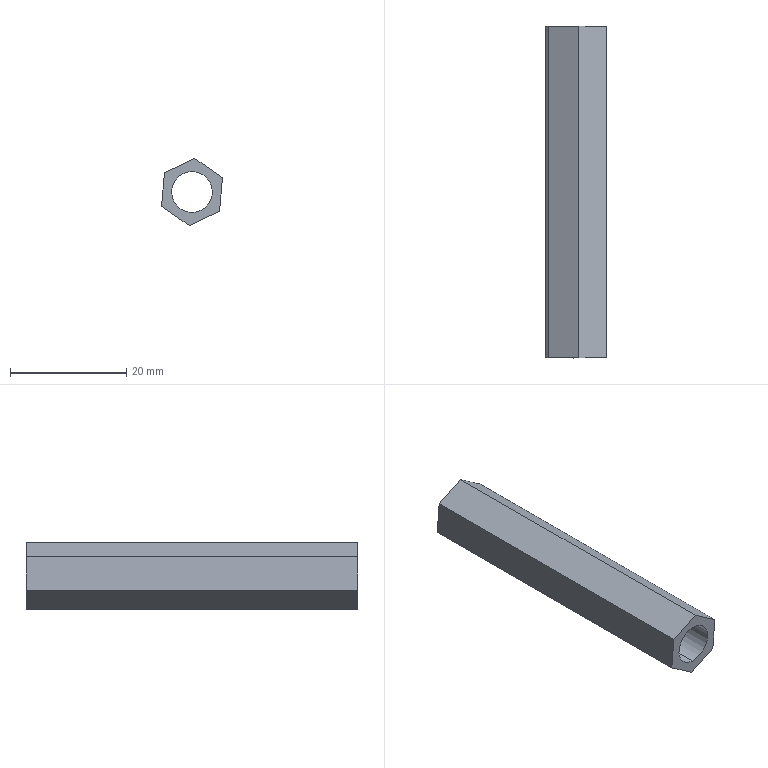Component | SolidWorks | HexagonalPost-1 | 1 solid | 10 faces | box 10.46 x 57 x 11.5 mm | volume 2743 mm3 | plane 8 | cylinder 2 | commonest cylinder face diameters 7 x2 | material Plain Carbon Steel
STEP:
#1=COLOUR_RGB('',0.7922,0.8196,0.9333);
#2=FILL_AREA_STYLE_COLOUR('',#1);
#3=FILL_AREA_STYLE('',(#2));
#4=SURFACE_STYLE_FILL_AREA(#3);
#5=SURFACE_SIDE_STYLE('',(#4));
#6=SURFACE_STYLE_USAGE(.BOTH.,#5);
#7=PRESENTATION_STYLE_ASSIGNMENT((#6));
#8=CARTESIAN_POINT('',(-177.617,347.975,291.332));
#9=VERTEX_POINT('',#8);
#10=CARTESIAN_POINT('',(-177.64,347.975,291.057));
#11=VERTEX_POINT('',#10);
#12=CARTESIAN_POINT('',(-177.628,347.975,291.195));
#13=DIRECTION('',(0.,1.,0.));
#14=DIRECTION('',(-0.08306,0.,-0.9965));
#15=AXIS2_PLACEMENT_3D('',#12,#13,#14);
#16=CIRCLE('',#15,0.1378);
#17=EDGE_CURVE('',#9,#11,#16,.T.);
#18=ORIENTED_EDGE('',*,*,#17,.T.);
#19=CARTESIAN_POINT('',(-177.64,345.731,291.057));
#20=VERTEX_POINT('',#19);
#21=CARTESIAN_POINT('',(-177.64,347.975,291.057));
#22=DIRECTION('',(-0.,-1.,-0.));
#23=VECTOR('',#22,39.37);
#24=LINE('',#21,#23);
#25=EDGE_CURVE('',#11,#20,#24,.T.);
#26=ORIENTED_EDGE('',*,*,#25,.T.);
#27=CARTESIAN_POINT('',(-177.617,345.731,291.332));
#28=VERTEX_POINT('',#27);
#29=CARTESIAN_POINT('',(-177.628,345.731,291.195));
#30=DIRECTION('',(0.,1.,0.));
#31=DIRECTION('',(-0.08306,0.,-0.9965));
#32=AXIS2_PLACEMENT_3D('',#29,#30,#31);
#33=CIRCLE('',#32,0.1378);
#34=EDGE_CURVE('',#28,#20,#33,.T.);
#35=ORIENTED_EDGE('',*,*,#34,.F.);
#36=CARTESIAN_POINT('',(-177.617,347.975,291.332));
#37=DIRECTION('',(-0.,-1.,-0.));
#38=VECTOR('',#37,39.37);
#39=LINE('',#36,#38);
#40=EDGE_CURVE('',#9,#28,#39,.T.);
#41=ORIENTED_EDGE('',*,*,#40,.F.);
#42=EDGE_LOOP('',(#18,#26,#35,#41));
#43=FACE_OUTER_BOUND('',#42,.T.);
#44=CARTESIAN_POINT('',(-177.628,347.975,291.195));
#45=DIRECTION('',(-0.,-1.,-0.));
#46=DIRECTION('',(0.08306,0.,0.9965));
#47=AXIS2_PLACEMENT_3D('',#44,#45,#46);
#48=CYLINDRICAL_SURFACE('',#47,0.1378);
#49=ADVANCED_FACE('',(#43),#48,.F.);
#50=CARTESIAN_POINT('',(-177.648,347.975,290.968));
#51=VERTEX_POINT('',#50);
#52=CARTESIAN_POINT('',(-177.834,347.975,291.098));
#53=VERTEX_POINT('',#52);
#54=CARTESIAN_POINT('',(-177.648,347.975,290.968));
#55=DIRECTION('',(-0.8199,0.,0.5726));
#56=VECTOR('',#55,39.37);
#57=LINE('',#54,#56);
#58=EDGE_CURVE('',#51,#53,#57,.T.);
#59=ORIENTED_EDGE('',*,*,#58,.T.);
#60=CARTESIAN_POINT('',(-177.815,347.975,291.325));
#61=VERTEX_POINT('',#60);
#62=CARTESIAN_POINT('',(-177.834,347.975,291.098));
#63=DIRECTION('',(0.08592,-0.,0.9963));
#64=VECTOR('',#63,39.37);
#65=LINE('',#62,#64);
#66=EDGE_CURVE('',#53,#61,#65,.T.);
#67=ORIENTED_EDGE('',*,*,#66,.T.);
#68=CARTESIAN_POINT('',(-177.609,347.975,291.421));
#69=VERTEX_POINT('',#68);
#70=CARTESIAN_POINT('',(-177.815,347.975,291.325));
#71=DIRECTION('',(0.9058,-0.,0.4237));
#72=VECTOR('',#71,39.37);
#73=LINE('',#70,#72);
#74=EDGE_CURVE('',#61,#69,#73,.T.);
#75=ORIENTED_EDGE('',*,*,#74,.T.);
#76=CARTESIAN_POINT('',(-177.422,347.975,291.291));
#77=VERTEX_POINT('',#76);
#78=CARTESIAN_POINT('',(-177.609,347.975,291.421));
#79=DIRECTION('',(0.8199,-0.,-0.5726));
#80=VECTOR('',#79,39.37);
#81=LINE('',#78,#80);
#82=EDGE_CURVE('',#69,#77,#81,.T.);
#83=ORIENTED_EDGE('',*,*,#82,.T.);
#84=CARTESIAN_POINT('',(-177.442,347.975,291.064));
#85=VERTEX_POINT('',#84);
#86=CARTESIAN_POINT('',(-177.422,347.975,291.291));
#87=DIRECTION('',(-0.08592,0.,-0.9963));
#88=VECTOR('',#87,39.37);
#89=LINE('',#86,#88);
#90=EDGE_CURVE('',#77,#85,#89,.T.);
#91=ORIENTED_EDGE('',*,*,#90,.T.);
#92=CARTESIAN_POINT('',(-177.442,347.975,291.064));
#93=DIRECTION('',(-0.9058,0.,-0.4237));
#94=VECTOR('',#93,39.37);
#95=LINE('',#92,#94);
#96=EDGE_CURVE('',#85,#51,#95,.T.);
#97=ORIENTED_EDGE('',*,*,#96,.T.);
#98=EDGE_LOOP('',(#59,#67,#75,#83,#91,#97));
#99=FACE_OUTER_BOUND('',#98,.T.);
#100=ORIENTED_EDGE('',*,*,#17,.F.);
#101=CARTESIAN_POINT('',(-177.628,347.975,291.195));
#102=DIRECTION('',(0.,1.,0.));
#103=DIRECTION('',(-0.08306,0.,-0.9965));
#104=AXIS2_PLACEMENT_3D('',#101,#102,#103);
#105=CIRCLE('',#104,0.1378);
#106=EDGE_CURVE('',#11,#9,#105,.T.);
#107=ORIENTED_EDGE('',*,*,#106,.F.);
#108=EDGE_LOOP('',(#100,#107));
#109=FACE_BOUND('',#108,.T.);
#110=CARTESIAN_POINT('',(-177.834,347.975,291.098));
#111=DIRECTION('',(0.,1.,0.));
#112=DIRECTION('',(-0.08306,0.,-0.9965));
#113=AXIS2_PLACEMENT_3D('',#110,#111,#112);
#114=PLANE('',#113);
#115=ADVANCED_FACE('',(#99,#109),#114,.T.);
#116=CARTESIAN_POINT('',(-177.648,345.731,290.968));
#117=VERTEX_POINT('',#116);
#118=CARTESIAN_POINT('',(-177.834,345.731,291.098));
#119=VERTEX_POINT('',#118);
#120=CARTESIAN_POINT('',(-177.648,345.731,290.968));
#121=DIRECTION('',(-0.8199,0.,0.5726));
#122=VECTOR('',#121,39.37);
#123=LINE('',#120,#122);
#124=EDGE_CURVE('',#117,#119,#123,.T.);
#125=ORIENTED_EDGE('',*,*,#124,.F.);
#126=CARTESIAN_POINT('',(-177.442,345.731,291.064));
#127=VERTEX_POINT('',#126);
#128=CARTESIAN_POINT('',(-177.442,345.731,291.064));
#129=DIRECTION('',(-0.9058,0.,-0.4237));
#130=VECTOR('',#129,39.37);
#131=LINE('',#128,#130);
#132=EDGE_CURVE('',#127,#117,#131,.T.);
#133=ORIENTED_EDGE('',*,*,#132,.F.);
#134=CARTESIAN_POINT('',(-177.422,345.731,291.291));
#135=VERTEX_POINT('',#134);
#136=CARTESIAN_POINT('',(-177.422,345.731,291.291));
#137=DIRECTION('',(-0.08592,0.,-0.9963));
#138=VECTOR('',#137,39.37);
#139=LINE('',#136,#138);
#140=EDGE_CURVE('',#135,#127,#139,.T.);
#141=ORIENTED_EDGE('',*,*,#140,.F.);
#142=CARTESIAN_POINT('',(-177.609,345.731,291.421));
#143=VERTEX_POINT('',#142);
#144=CARTESIAN_POINT('',(-177.609,345.731,291.421));
#145=DIRECTION('',(0.8199,-0.,-0.5726));
#146=VECTOR('',#145,39.37);
#147=LINE('',#144,#146);
#148=EDGE_CURVE('',#143,#135,#147,.T.);
#149=ORIENTED_EDGE('',*,*,#148,.F.);
#150=CARTESIAN_POINT('',(-177.815,345.731,291.325));
#151=VERTEX_POINT('',#150);
#152=CARTESIAN_POINT('',(-177.815,345.731,291.325));
#153=DIRECTION('',(0.9058,-0.,0.4237));
#154=VECTOR('',#153,39.37);
#155=LINE('',#152,#154);
#156=EDGE_CURVE('',#151,#143,#155,.T.);
#157=ORIENTED_EDGE('',*,*,#156,.F.);
#158=CARTESIAN_POINT('',(-177.834,345.731,291.098));
#159=DIRECTION('',(0.08592,-0.,0.9963));
#160=VECTOR('',#159,39.37);
#161=LINE('',#158,#160);
#162=EDGE_CURVE('',#119,#151,#161,.T.);
#163=ORIENTED_EDGE('',*,*,#162,.F.);
#164=EDGE_LOOP('',(#125,#133,#141,#149,#157,#163));
#165=FACE_OUTER_BOUND('',#164,.T.);
#166=ORIENTED_EDGE('',*,*,#34,.T.);
#167=CARTESIAN_POINT('',(-177.628,345.731,291.195));
#168=DIRECTION('',(0.,1.,0.));
#169=DIRECTION('',(-0.08306,0.,-0.9965));
#170=AXIS2_PLACEMENT_3D('',#167,#168,#169);
#171=CIRCLE('',#170,0.1378);
#172=EDGE_CURVE('',#20,#28,#171,.T.);
#173=ORIENTED_EDGE('',*,*,#172,.T.);
#174=EDGE_LOOP('',(#166,#173));
#175=FACE_BOUND('',#174,.T.);
#176=CARTESIAN_POINT('',(-177.834,345.731,291.098));
#177=DIRECTION('',(0.,1.,0.));
#178=DIRECTION('',(-0.08306,0.,-0.9965));
#179=AXIS2_PLACEMENT_3D('',#176,#177,#178);
#180=PLANE('',#179);
#181=ADVANCED_FACE('',(#165,#175),#180,.F.);
#182=ORIENTED_EDGE('',*,*,#124,.T.);
#183=CARTESIAN_POINT('',(-177.834,347.975,291.098));
#184=DIRECTION('',(-0.,-1.,-0.));
#185=VECTOR('',#184,39.37);
#186=LINE('',#183,#185);
#187=EDGE_CURVE('',#53,#119,#186,.T.);
#188=ORIENTED_EDGE('',*,*,#187,.F.);
#189=ORIENTED_EDGE('',*,*,#58,.F.);
#190=CARTESIAN_POINT('',(-177.648,347.975,290.968));
#191=DIRECTION('',(-0.,-1.,-0.));
#192=VECTOR('',#191,39.37);
#193=LINE('',#190,#192);
#194=EDGE_CURVE('',#51,#117,#193,.T.);
#195=ORIENTED_EDGE('',*,*,#194,.T.);
#196=EDGE_LOOP('',(#182,#188,#189,#195));
#197=FACE_OUTER_BOUND('',#196,.T.);
#198=CARTESIAN_POINT('',(-177.648,347.975,290.968));
#199=DIRECTION('',(0.5726,-0.,0.8199));
#200=DIRECTION('',(0.8199,-0.,-0.5726));
#201=AXIS2_PLACEMENT_3D('',#198,#199,#200);
#202=PLANE('',#201);
#203=ADVANCED_FACE('',(#197),#202,.F.);
#204=ORIENTED_EDGE('',*,*,#162,.T.);
#205=CARTESIAN_POINT('',(-177.815,347.975,291.325));
#206=DIRECTION('',(-0.,-1.,-0.));
#207=VECTOR('',#206,39.37);
#208=LINE('',#205,#207);
#209=EDGE_CURVE('',#61,#151,#208,.T.);
#210=ORIENTED_EDGE('',*,*,#209,.F.);
#211=ORIENTED_EDGE('',*,*,#66,.F.);
#212=ORIENTED_EDGE('',*,*,#187,.T.);
#213=EDGE_LOOP('',(#204,#210,#211,#212));
#214=FACE_OUTER_BOUND('',#213,.T.);
#215=CARTESIAN_POINT('',(-177.834,347.975,291.098));
#216=DIRECTION('',(0.9963,-0.,-0.08592));
#217=DIRECTION('',(-0.08592,0.,-0.9963));
#218=AXIS2_PLACEMENT_3D('',#215,#216,#217);
#219=PLANE('',#218);
#220=ADVANCED_FACE('',(#214),#219,.F.);
#221=ORIENTED_EDGE('',*,*,#156,.T.);
#222=CARTESIAN_POINT('',(-177.609,347.975,291.421));
#223=DIRECTION('',(-0.,-1.,-0.));
#224=VECTOR('',#223,39.37);
#225=LINE('',#222,#224);
#226=EDGE_CURVE('',#69,#143,#225,.T.);
#227=ORIENTED_EDGE('',*,*,#226,.F.);
#228=ORIENTED_EDGE('',*,*,#74,.F.);
#229=ORIENTED_EDGE('',*,*,#209,.T.);
#230=EDGE_LOOP('',(#221,#227,#228,#229));
#231=FACE_OUTER_BOUND('',#230,.T.);
#232=CARTESIAN_POINT('',(-177.815,347.975,291.325));
#233=DIRECTION('',(0.4237,-0.,-0.9058));
#234=DIRECTION('',(-0.9058,0.,-0.4237));
#235=AXIS2_PLACEMENT_3D('',#232,#233,#234);
#236=PLANE('',#235);
#237=ADVANCED_FACE('',(#231),#236,.F.);
#238=ORIENTED_EDGE('',*,*,#148,.T.);
#239=CARTESIAN_POINT('',(-177.422,347.975,291.291));
#240=DIRECTION('',(-0.,-1.,-0.));
#241=VECTOR('',#240,39.37);
#242=LINE('',#239,#241);
#243=EDGE_CURVE('',#77,#135,#242,.T.);
#244=ORIENTED_EDGE('',*,*,#243,.F.);
#245=ORIENTED_EDGE('',*,*,#82,.F.);
#246=ORIENTED_EDGE('',*,*,#226,.T.);
#247=EDGE_LOOP('',(#238,#244,#245,#246));
#248=FACE_OUTER_BOUND('',#247,.T.);
#249=CARTESIAN_POINT('',(-177.609,347.975,291.421));
#250=DIRECTION('',(-0.5726,0.,-0.8199));
#251=DIRECTION('',(-0.8199,0.,0.5726));
#252=AXIS2_PLACEMENT_3D('',#249,#250,#251);
#253=PLANE('',#252);
#254=ADVANCED_FACE('',(#248),#253,.F.);
#255=ORIENTED_EDGE('',*,*,#140,.T.);
#256=CARTESIAN_POINT('',(-177.442,347.975,291.064));
#257=DIRECTION('',(-0.,-1.,-0.));
#258=VECTOR('',#257,39.37);
#259=LINE('',#256,#258);
#260=EDGE_CURVE('',#85,#127,#259,.T.);
#261=ORIENTED_EDGE('',*,*,#260,.F.);
#262=ORIENTED_EDGE('',*,*,#90,.F.);
#263=ORIENTED_EDGE('',*,*,#243,.T.);
#264=EDGE_LOOP('',(#255,#261,#262,#263));
#265=FACE_OUTER_BOUND('',#264,.T.);
#266=CARTESIAN_POINT('',(-177.422,347.975,291.291));
#267=DIRECTION('',(-0.9963,0.,0.08592));
#268=DIRECTION('',(0.08592,-0.,0.9963));
#269=AXIS2_PLACEMENT_3D('',#266,#267,#268);
#270=PLANE('',#269);
#271=ADVANCED_FACE('',(#265),#270,.F.);
#272=ORIENTED_EDGE('',*,*,#132,.T.);
#273=ORIENTED_EDGE('',*,*,#194,.F.);
#274=ORIENTED_EDGE('',*,*,#96,.F.);
#275=ORIENTED_EDGE('',*,*,#260,.T.);
#276=EDGE_LOOP('',(#272,#273,#274,#275));
#277=FACE_OUTER_BOUND('',#276,.T.);
#278=CARTESIAN_POINT('',(-177.442,347.975,291.064));
#279=DIRECTION('',(-0.4237,0.,0.9058));
#280=DIRECTION('',(0.9058,-0.,0.4237));
#281=AXIS2_PLACEMENT_3D('',#278,#279,#280);
#282=PLANE('',#281);
#283=ADVANCED_FACE('',(#277),#282,.F.);
#284=ORIENTED_EDGE('',*,*,#25,.F.);
#285=ORIENTED_EDGE('',*,*,#106,.T.);
#286=ORIENTED_EDGE('',*,*,#40,.T.);
#287=ORIENTED_EDGE('',*,*,#172,.F.);
#288=EDGE_LOOP('',(#284,#285,#286,#287));
#289=FACE_OUTER_BOUND('',#288,.T.);
#290=CARTESIAN_POINT('',(-177.628,347.975,291.195));
#291=DIRECTION('',(-0.,-1.,-0.));
#292=DIRECTION('',(0.08306,0.,0.9965));
#293=AXIS2_PLACEMENT_3D('',#290,#291,#292);
#294=CYLINDRICAL_SURFACE('',#293,0.1378);
#295=ADVANCED_FACE('',(#289),#294,.F.);
#296=CLOSED_SHELL('',(#49,#115,#181,#203,#220,#237,#254,#271,#283,#295));
#297=MANIFOLD_SOLID_BREP('',#296);
#298=STYLED_ITEM('',(#7),#297);
#299=(LENGTH_UNIT()NAMED_UNIT(*)SI_UNIT($,.METRE.));
#300=LENGTH_MEASURE_WITH_UNIT(LENGTH_MEASURE(0.0254),#299);
#301=DIMENSIONAL_EXPONENTS(1.,0.,0.,0.,0.,0.,0.);
#302=(CONVERSION_BASED_UNIT('',#300)LENGTH_UNIT()NAMED_UNIT(#301));
#303=UNCERTAINTY_MEASURE_WITH_UNIT(LENGTH_MEASURE(0.00001),#302,'','');
#304=(NAMED_UNIT(*)PLANE_ANGLE_UNIT()SI_UNIT($,.RADIAN.));
#305=(NAMED_UNIT(*)SI_UNIT($,.STERADIAN.)SOLID_ANGLE_UNIT());
#306=(GEOMETRIC_REPRESENTATION_CONTEXT(3)GLOBAL_UNCERTAINTY_ASSIGNED_CONTEXT((#303))GLOBAL_UNIT_ASSIGNED_CONTEXT((#302,#304,#305))REPRESENTATION_CONTEXT('',''));
#307=MECHANICAL_DESIGN_GEOMETRIC_PRESENTATION_REPRESENTATION('',(#298),#306);
#308=PRESENTATION_LAYER_ASSIGNMENT('','',(#298));
#309=CARTESIAN_POINT('',(0.,0.,0.));
#310=DIRECTION('',(0.,0.,1.));
#311=DIRECTION('',(1.,0.,0.));
#312=AXIS2_PLACEMENT_3D('',#309,#310,#311);
#313=(LENGTH_UNIT()NAMED_UNIT(*)SI_UNIT($,.METRE.));
#314=LENGTH_MEASURE_WITH_UNIT(LENGTH_MEASURE(0.0254),#313);
#315=DIMENSIONAL_EXPONENTS(1.,0.,0.,0.,0.,0.,0.);
#316=(CONVERSION_BASED_UNIT('',#314)LENGTH_UNIT()NAMED_UNIT(#315));
#317=UNCERTAINTY_MEASURE_WITH_UNIT(LENGTH_MEASURE(0.00001),#316,'','');
#318=(NAMED_UNIT(*)PLANE_ANGLE_UNIT()SI_UNIT($,.RADIAN.));
#319=(NAMED_UNIT(*)SI_UNIT($,.STERADIAN.)SOLID_ANGLE_UNIT());
#320=(GEOMETRIC_REPRESENTATION_CONTEXT(3)GLOBAL_UNCERTAINTY_ASSIGNED_CONTEXT((#317))GLOBAL_UNIT_ASSIGNED_CONTEXT((#316,#318,#319))REPRESENTATION_CONTEXT('',''));
#321=ADVANCED_BREP_SHAPE_REPRESENTATION('',(#297,#312),#320);